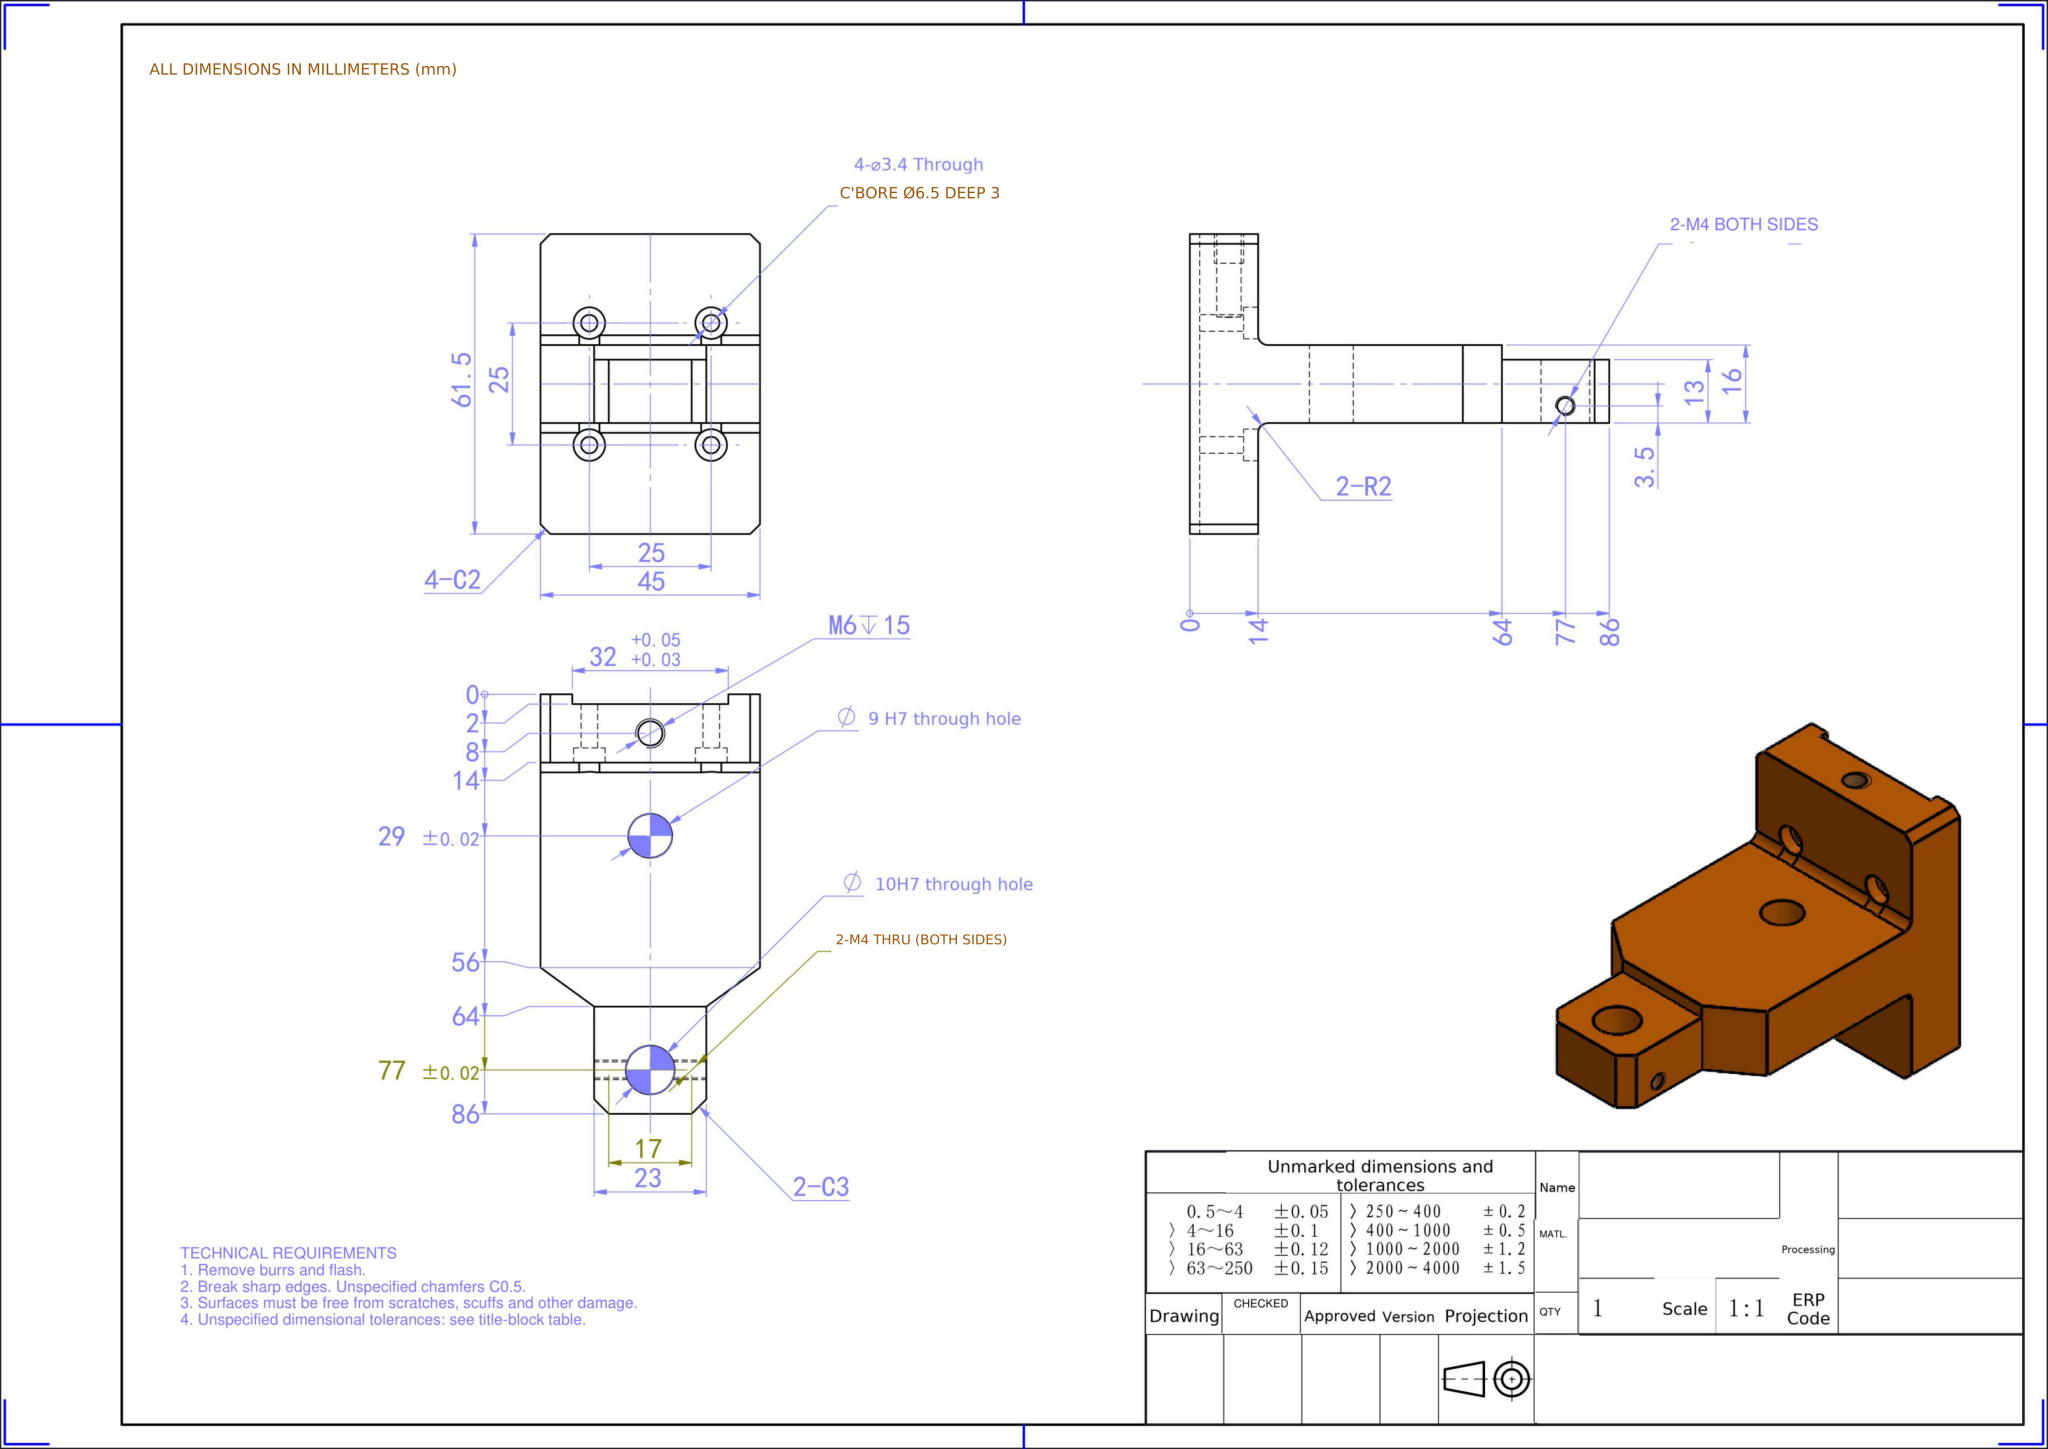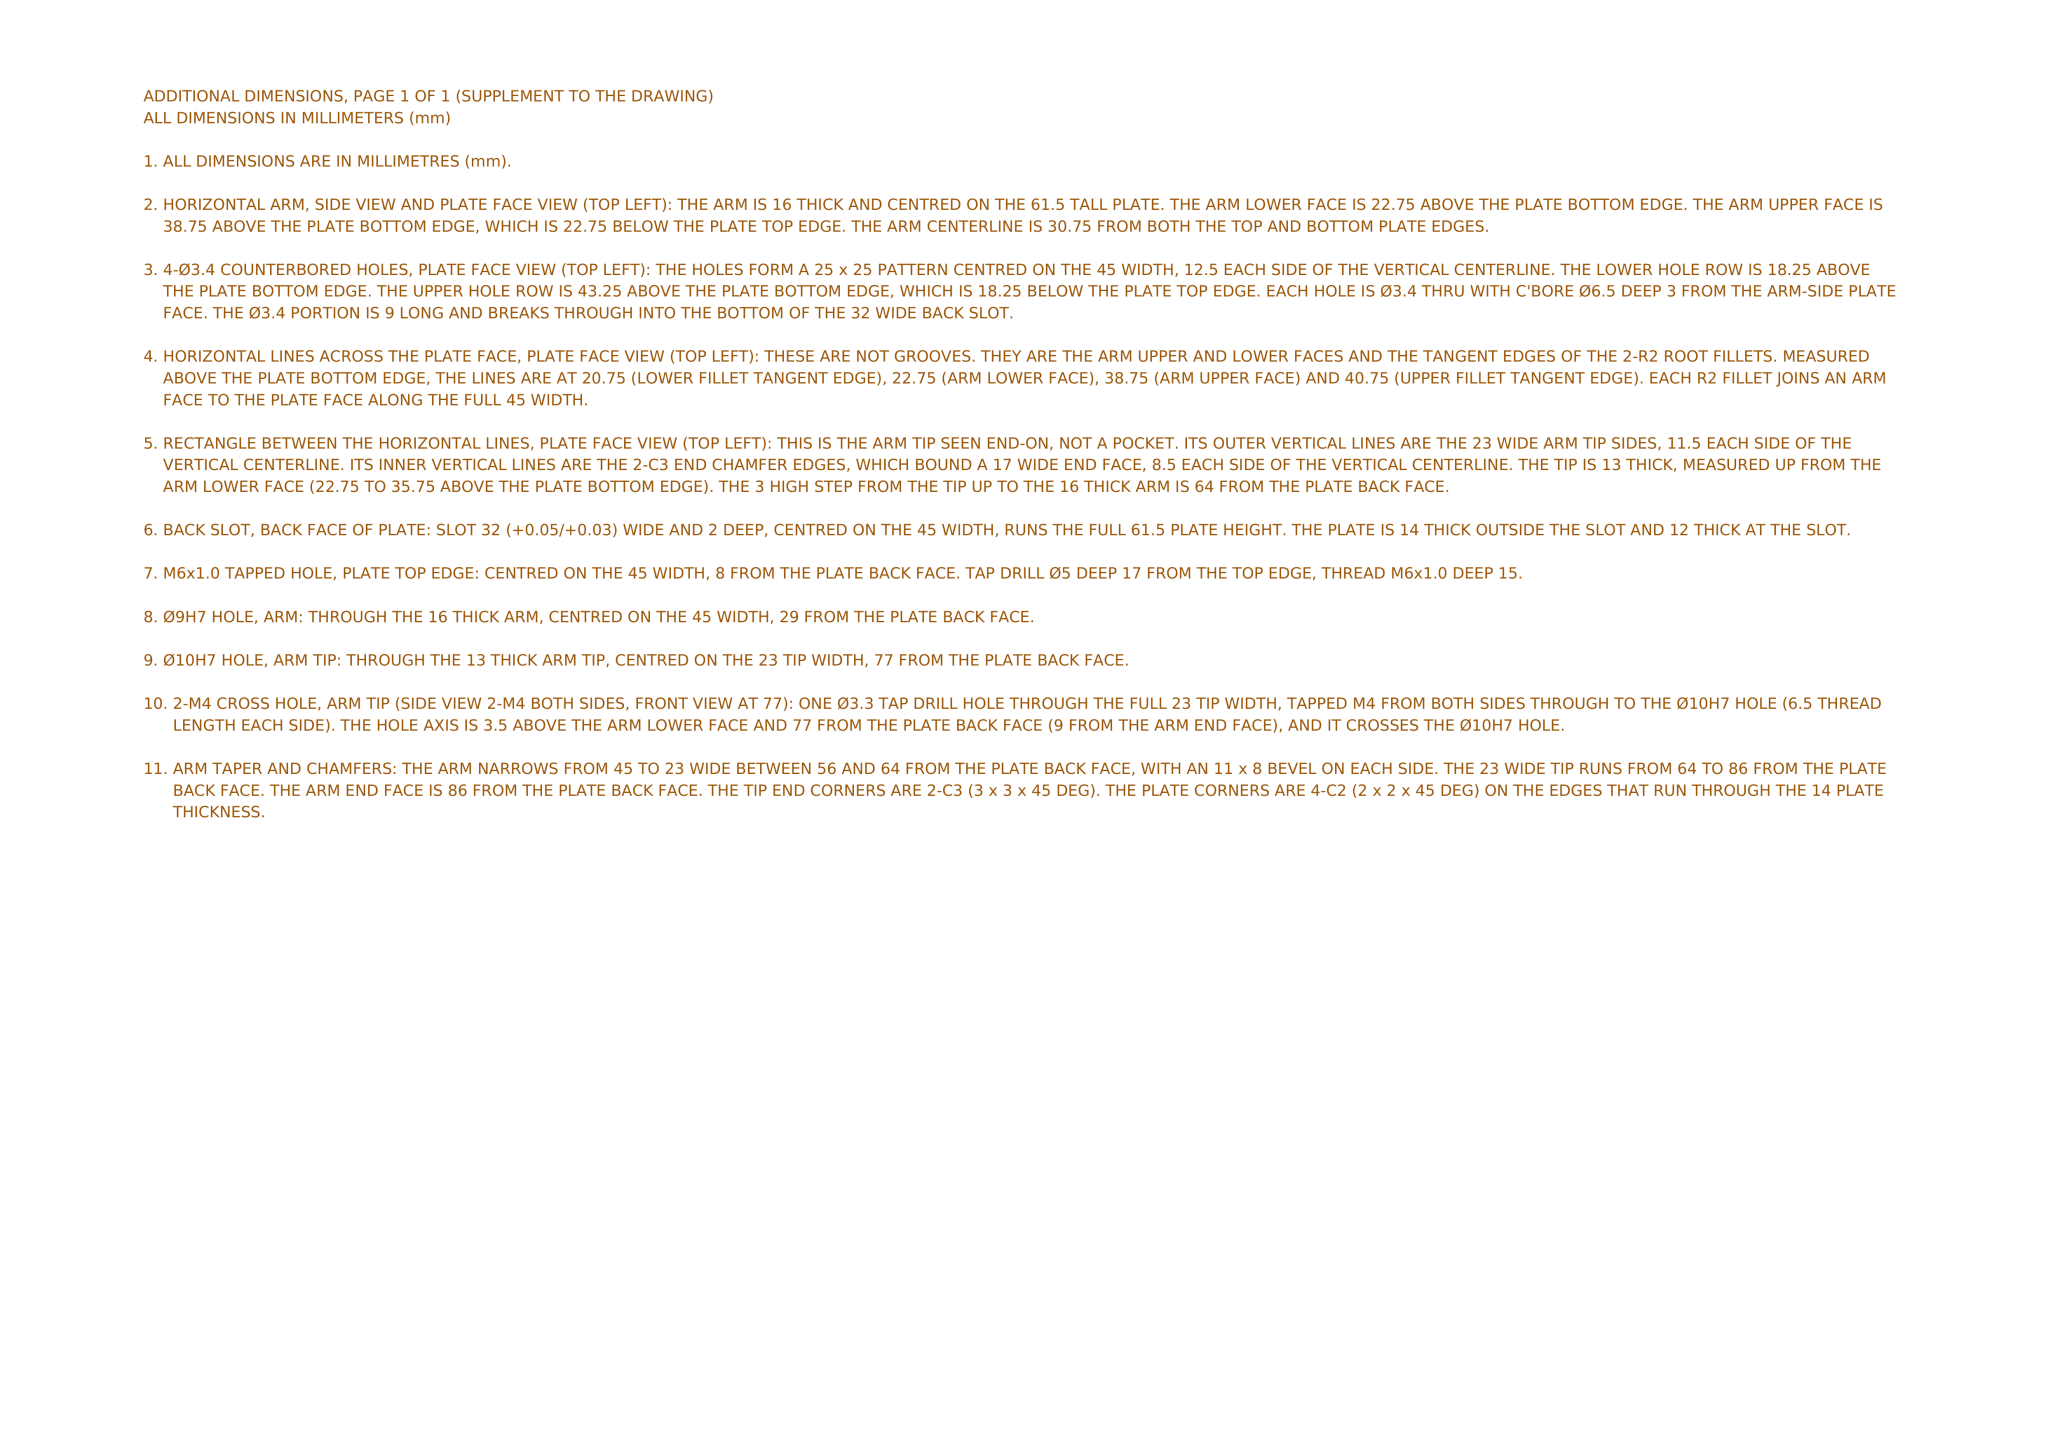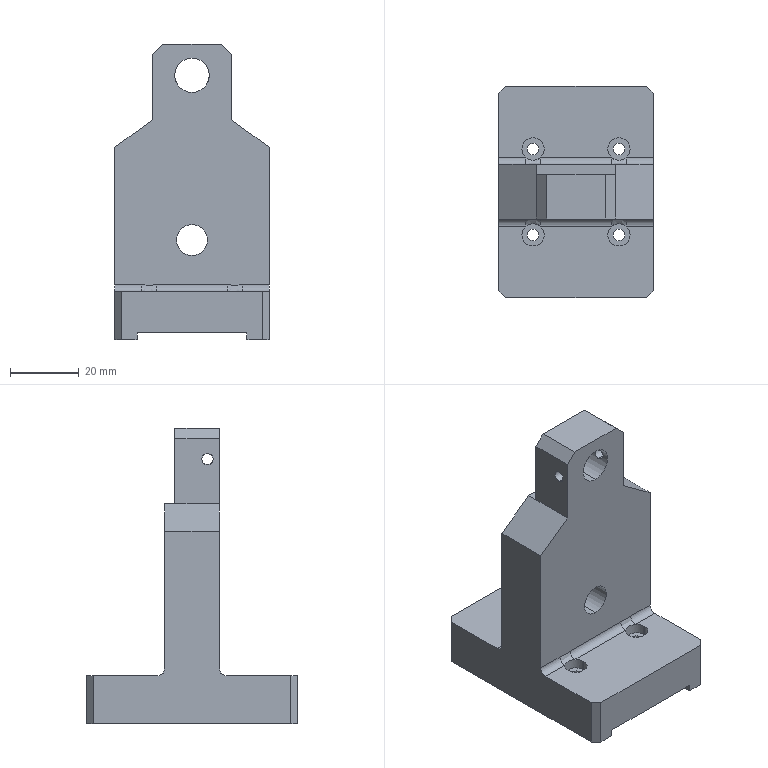Part | NX | mm | 1 solid | 68 faces | box 45 x 61.5 x 86 mm | volume 72614 mm3 | cylinder 32 | plane 30 | spline 4 | cone 2 | commonest cylinder face diameters 6.5 x8 3.4 x8 4 x6 3.3 x4 5 x2 9 x2 10 x2